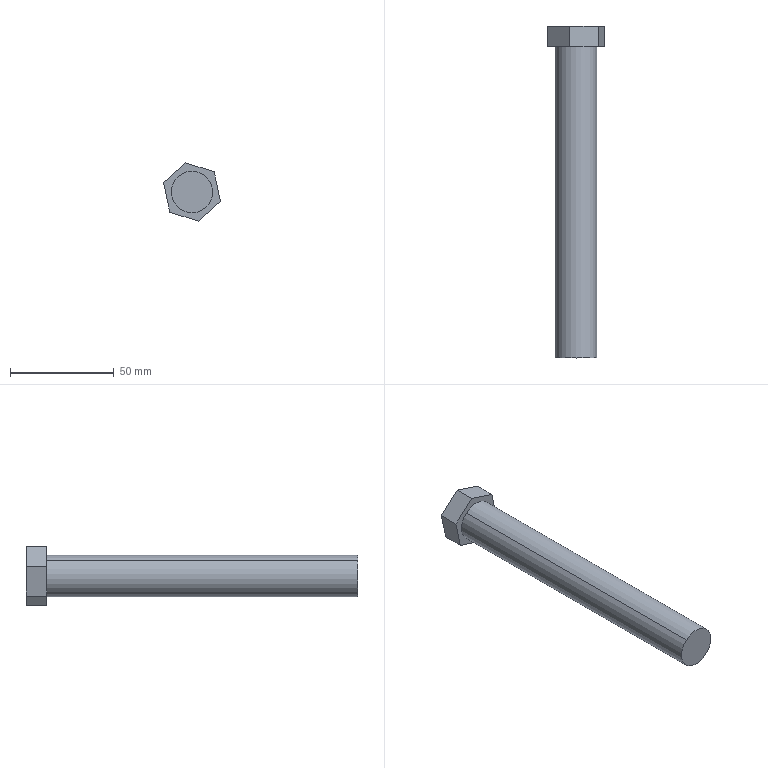Component | SolidWorks | -LimitScrewRod-1 | 1 solid | 11 faces | box 27.46 x 160 x 28.24 mm | volume 52537 mm3 | plane 9 | cylinder 2 | commonest cylinder face diameters 20 x2
STEP:
#1=COLOUR_RGB('',0.7922,0.8196,0.9333);
#2=FILL_AREA_STYLE_COLOUR('',#1);
#3=FILL_AREA_STYLE('',(#2));
#4=SURFACE_STYLE_FILL_AREA(#3);
#5=SURFACE_SIDE_STYLE('',(#4));
#6=SURFACE_STYLE_USAGE(.BOTH.,#5);
#7=PRESENTATION_STYLE_ASSIGNMENT((#6));
#8=CARTESIAN_POINT('',(0.9176,41.772,-4.432));
#9=VERTEX_POINT('',#8);
#10=CARTESIAN_POINT('',(1.445,41.772,-5.017));
#11=VERTEX_POINT('',#10);
#12=CARTESIAN_POINT('',(1.181,41.772,-4.724));
#13=DIRECTION('',(0.,-1.,0.));
#14=DIRECTION('',(-0.6693,0.,0.743));
#15=AXIS2_PLACEMENT_3D('',#12,#13,#14);
#16=CIRCLE('',#15,0.3937);
#17=EDGE_CURVE('',#9,#11,#16,.T.);
#18=ORIENTED_EDGE('',*,*,#17,.F.);
#19=CARTESIAN_POINT('',(0.9176,47.677,-4.432));
#20=VERTEX_POINT('',#19);
#21=CARTESIAN_POINT('',(0.9176,41.772,-4.432));
#22=DIRECTION('',(0.,1.,0.));
#23=VECTOR('',#22,39.37);
#24=LINE('',#21,#23);
#25=EDGE_CURVE('',#9,#20,#24,.T.);
#26=ORIENTED_EDGE('',*,*,#25,.T.);
#27=CARTESIAN_POINT('',(1.445,47.677,-5.017));
#28=VERTEX_POINT('',#27);
#29=CARTESIAN_POINT('',(1.181,47.677,-4.724));
#30=DIRECTION('',(0.,-1.,0.));
#31=DIRECTION('',(-0.6693,0.,0.743));
#32=AXIS2_PLACEMENT_3D('',#29,#30,#31);
#33=CIRCLE('',#32,0.3937);
#34=EDGE_CURVE('',#20,#28,#33,.T.);
#35=ORIENTED_EDGE('',*,*,#34,.T.);
#36=CARTESIAN_POINT('',(1.445,41.772,-5.017));
#37=DIRECTION('',(0.,1.,0.));
#38=VECTOR('',#37,39.37);
#39=LINE('',#36,#38);
#40=EDGE_CURVE('',#11,#28,#39,.T.);
#41=ORIENTED_EDGE('',*,*,#40,.F.);
#42=EDGE_LOOP('',(#18,#26,#35,#41));
#43=FACE_OUTER_BOUND('',#42,.T.);
#44=CARTESIAN_POINT('',(1.181,41.772,-4.724));
#45=DIRECTION('',(0.,1.,0.));
#46=DIRECTION('',(0.6693,0.,-0.743));
#47=AXIS2_PLACEMENT_3D('',#44,#45,#46);
#48=CYLINDRICAL_SURFACE('',#47,0.3937);
#49=ADVANCED_FACE('',(#43),#48,.T.);
#50=CARTESIAN_POINT('',(0.6406,47.677,-4.549));
#51=VERTEX_POINT('',#50);
#52=CARTESIAN_POINT('',(0.7589,47.677,-5.105));
#53=VERTEX_POINT('',#52);
#54=CARTESIAN_POINT('',(0.6406,47.677,-4.549));
#55=DIRECTION('',(0.2081,0.,-0.9781));
#56=VECTOR('',#55,39.37);
#57=LINE('',#54,#56);
#58=EDGE_CURVE('',#51,#53,#57,.T.);
#59=ORIENTED_EDGE('',*,*,#58,.T.);
#60=CARTESIAN_POINT('',(1.299,47.677,-5.28));
#61=VERTEX_POINT('',#60);
#62=CARTESIAN_POINT('',(0.7589,47.677,-5.105));
#63=DIRECTION('',(0.9511,0.,-0.3088));
#64=VECTOR('',#63,39.37);
#65=LINE('',#62,#64);
#66=EDGE_CURVE('',#53,#61,#65,.T.);
#67=ORIENTED_EDGE('',*,*,#66,.T.);
#68=CARTESIAN_POINT('',(1.722,47.677,-4.9));
#69=VERTEX_POINT('',#68);
#70=CARTESIAN_POINT('',(1.299,47.677,-5.28));
#71=DIRECTION('',(0.743,0.,0.6693));
#72=VECTOR('',#71,39.37);
#73=LINE('',#70,#72);
#74=EDGE_CURVE('',#61,#69,#73,.T.);
#75=ORIENTED_EDGE('',*,*,#74,.T.);
#76=CARTESIAN_POINT('',(1.603,47.677,-4.344));
#77=VERTEX_POINT('',#76);
#78=CARTESIAN_POINT('',(1.722,47.677,-4.9));
#79=DIRECTION('',(-0.2081,0.,0.9781));
#80=VECTOR('',#79,39.37);
#81=LINE('',#78,#80);
#82=EDGE_CURVE('',#69,#77,#81,.T.);
#83=ORIENTED_EDGE('',*,*,#82,.T.);
#84=CARTESIAN_POINT('',(1.063,47.677,-4.169));
#85=VERTEX_POINT('',#84);
#86=CARTESIAN_POINT('',(1.603,47.677,-4.344));
#87=DIRECTION('',(-0.9511,0.,0.3088));
#88=VECTOR('',#87,39.37);
#89=LINE('',#86,#88);
#90=EDGE_CURVE('',#77,#85,#89,.T.);
#91=ORIENTED_EDGE('',*,*,#90,.T.);
#92=CARTESIAN_POINT('',(1.063,47.677,-4.169));
#93=DIRECTION('',(-0.743,0.,-0.6693));
#94=VECTOR('',#93,39.37);
#95=LINE('',#92,#94);
#96=EDGE_CURVE('',#85,#51,#95,.T.);
#97=ORIENTED_EDGE('',*,*,#96,.T.);
#98=EDGE_LOOP('',(#59,#67,#75,#83,#91,#97));
#99=FACE_OUTER_BOUND('',#98,.T.);
#100=CARTESIAN_POINT('',(1.181,47.677,-4.724));
#101=DIRECTION('',(0.,-1.,0.));
#102=DIRECTION('',(-0.6693,0.,0.743));
#103=AXIS2_PLACEMENT_3D('',#100,#101,#102);
#104=CIRCLE('',#103,0.3937);
#105=EDGE_CURVE('',#28,#20,#104,.T.);
#106=ORIENTED_EDGE('',*,*,#105,.F.);
#107=ORIENTED_EDGE('',*,*,#34,.F.);
#108=EDGE_LOOP('',(#106,#107));
#109=FACE_BOUND('',#108,.T.);
#110=CARTESIAN_POINT('',(1.181,47.677,-4.724));
#111=DIRECTION('',(0.,-1.,0.));
#112=DIRECTION('',(-0.6693,0.,0.743));
#113=AXIS2_PLACEMENT_3D('',#110,#111,#112);
#114=PLANE('',#113);
#115=ADVANCED_FACE('',(#99,#109),#114,.T.);
#116=CARTESIAN_POINT('',(0.6406,48.071,-4.549));
#117=VERTEX_POINT('',#116);
#118=CARTESIAN_POINT('',(0.7589,48.071,-5.105));
#119=VERTEX_POINT('',#118);
#120=CARTESIAN_POINT('',(0.6406,48.071,-4.549));
#121=DIRECTION('',(0.2081,0.,-0.9781));
#122=VECTOR('',#121,39.37);
#123=LINE('',#120,#122);
#124=EDGE_CURVE('',#117,#119,#123,.T.);
#125=ORIENTED_EDGE('',*,*,#124,.T.);
#126=CARTESIAN_POINT('',(0.7589,47.677,-5.105));
#127=DIRECTION('',(0.,1.,0.));
#128=VECTOR('',#127,39.37);
#129=LINE('',#126,#128);
#130=EDGE_CURVE('',#53,#119,#129,.T.);
#131=ORIENTED_EDGE('',*,*,#130,.F.);
#132=ORIENTED_EDGE('',*,*,#58,.F.);
#133=CARTESIAN_POINT('',(0.6406,47.677,-4.549));
#134=DIRECTION('',(0.,1.,0.));
#135=VECTOR('',#134,39.37);
#136=LINE('',#133,#135);
#137=EDGE_CURVE('',#51,#117,#136,.T.);
#138=ORIENTED_EDGE('',*,*,#137,.T.);
#139=EDGE_LOOP('',(#125,#131,#132,#138));
#140=FACE_OUTER_BOUND('',#139,.T.);
#141=CARTESIAN_POINT('',(0.6406,47.677,-4.549));
#142=DIRECTION('',(0.9781,0.,0.2081));
#143=DIRECTION('',(-0.2081,0.,0.9781));
#144=AXIS2_PLACEMENT_3D('',#141,#142,#143);
#145=PLANE('',#144);
#146=ADVANCED_FACE('',(#140),#145,.F.);
#147=CARTESIAN_POINT('',(1.299,48.071,-5.28));
#148=VERTEX_POINT('',#147);
#149=CARTESIAN_POINT('',(0.7589,48.071,-5.105));
#150=DIRECTION('',(0.9511,0.,-0.3088));
#151=VECTOR('',#150,39.37);
#152=LINE('',#149,#151);
#153=EDGE_CURVE('',#119,#148,#152,.T.);
#154=ORIENTED_EDGE('',*,*,#153,.T.);
#155=CARTESIAN_POINT('',(1.299,47.677,-5.28));
#156=DIRECTION('',(0.,1.,0.));
#157=VECTOR('',#156,39.37);
#158=LINE('',#155,#157);
#159=EDGE_CURVE('',#61,#148,#158,.T.);
#160=ORIENTED_EDGE('',*,*,#159,.F.);
#161=ORIENTED_EDGE('',*,*,#66,.F.);
#162=ORIENTED_EDGE('',*,*,#130,.T.);
#163=EDGE_LOOP('',(#154,#160,#161,#162));
#164=FACE_OUTER_BOUND('',#163,.T.);
#165=CARTESIAN_POINT('',(0.7589,47.677,-5.105));
#166=DIRECTION('',(0.3088,0.,0.9511));
#167=DIRECTION('',(-0.9511,0.,0.3088));
#168=AXIS2_PLACEMENT_3D('',#165,#166,#167);
#169=PLANE('',#168);
#170=ADVANCED_FACE('',(#164),#169,.F.);
#171=CARTESIAN_POINT('',(1.722,48.071,-4.9));
#172=VERTEX_POINT('',#171);
#173=CARTESIAN_POINT('',(1.299,48.071,-5.28));
#174=DIRECTION('',(0.743,0.,0.6693));
#175=VECTOR('',#174,39.37);
#176=LINE('',#173,#175);
#177=EDGE_CURVE('',#148,#172,#176,.T.);
#178=ORIENTED_EDGE('',*,*,#177,.T.);
#179=CARTESIAN_POINT('',(1.722,47.677,-4.9));
#180=DIRECTION('',(0.,1.,0.));
#181=VECTOR('',#180,39.37);
#182=LINE('',#179,#181);
#183=EDGE_CURVE('',#69,#172,#182,.T.);
#184=ORIENTED_EDGE('',*,*,#183,.F.);
#185=ORIENTED_EDGE('',*,*,#74,.F.);
#186=ORIENTED_EDGE('',*,*,#159,.T.);
#187=EDGE_LOOP('',(#178,#184,#185,#186));
#188=FACE_OUTER_BOUND('',#187,.T.);
#189=CARTESIAN_POINT('',(1.299,47.677,-5.28));
#190=DIRECTION('',(-0.6693,0.,0.743));
#191=DIRECTION('',(-0.743,0.,-0.6693));
#192=AXIS2_PLACEMENT_3D('',#189,#190,#191);
#193=PLANE('',#192);
#194=ADVANCED_FACE('',(#188),#193,.F.);
#195=CARTESIAN_POINT('',(1.603,48.071,-4.344));
#196=VERTEX_POINT('',#195);
#197=CARTESIAN_POINT('',(1.722,48.071,-4.9));
#198=DIRECTION('',(-0.2081,0.,0.9781));
#199=VECTOR('',#198,39.37);
#200=LINE('',#197,#199);
#201=EDGE_CURVE('',#172,#196,#200,.T.);
#202=ORIENTED_EDGE('',*,*,#201,.T.);
#203=CARTESIAN_POINT('',(1.603,47.677,-4.344));
#204=DIRECTION('',(0.,1.,0.));
#205=VECTOR('',#204,39.37);
#206=LINE('',#203,#205);
#207=EDGE_CURVE('',#77,#196,#206,.T.);
#208=ORIENTED_EDGE('',*,*,#207,.F.);
#209=ORIENTED_EDGE('',*,*,#82,.F.);
#210=ORIENTED_EDGE('',*,*,#183,.T.);
#211=EDGE_LOOP('',(#202,#208,#209,#210));
#212=FACE_OUTER_BOUND('',#211,.T.);
#213=CARTESIAN_POINT('',(1.722,47.677,-4.9));
#214=DIRECTION('',(-0.9781,0.,-0.2081));
#215=DIRECTION('',(0.2081,0.,-0.9781));
#216=AXIS2_PLACEMENT_3D('',#213,#214,#215);
#217=PLANE('',#216);
#218=ADVANCED_FACE('',(#212),#217,.F.);
#219=CARTESIAN_POINT('',(1.063,48.071,-4.169));
#220=VERTEX_POINT('',#219);
#221=CARTESIAN_POINT('',(1.603,48.071,-4.344));
#222=DIRECTION('',(-0.9511,0.,0.3088));
#223=VECTOR('',#222,39.37);
#224=LINE('',#221,#223);
#225=EDGE_CURVE('',#196,#220,#224,.T.);
#226=ORIENTED_EDGE('',*,*,#225,.T.);
#227=CARTESIAN_POINT('',(1.063,47.677,-4.169));
#228=DIRECTION('',(0.,1.,0.));
#229=VECTOR('',#228,39.37);
#230=LINE('',#227,#229);
#231=EDGE_CURVE('',#85,#220,#230,.T.);
#232=ORIENTED_EDGE('',*,*,#231,.F.);
#233=ORIENTED_EDGE('',*,*,#90,.F.);
#234=ORIENTED_EDGE('',*,*,#207,.T.);
#235=EDGE_LOOP('',(#226,#232,#233,#234));
#236=FACE_OUTER_BOUND('',#235,.T.);
#237=CARTESIAN_POINT('',(1.603,47.677,-4.344));
#238=DIRECTION('',(-0.3088,0.,-0.9511));
#239=DIRECTION('',(0.9511,0.,-0.3088));
#240=AXIS2_PLACEMENT_3D('',#237,#238,#239);
#241=PLANE('',#240);
#242=ADVANCED_FACE('',(#236),#241,.F.);
#243=CARTESIAN_POINT('',(1.063,48.071,-4.169));
#244=DIRECTION('',(-0.743,0.,-0.6693));
#245=VECTOR('',#244,39.37);
#246=LINE('',#243,#245);
#247=EDGE_CURVE('',#220,#117,#246,.T.);
#248=ORIENTED_EDGE('',*,*,#247,.T.);
#249=ORIENTED_EDGE('',*,*,#137,.F.);
#250=ORIENTED_EDGE('',*,*,#96,.F.);
#251=ORIENTED_EDGE('',*,*,#231,.T.);
#252=EDGE_LOOP('',(#248,#249,#250,#251));
#253=FACE_OUTER_BOUND('',#252,.T.);
#254=CARTESIAN_POINT('',(1.063,47.677,-4.169));
#255=DIRECTION('',(0.6693,0.,-0.743));
#256=DIRECTION('',(0.743,0.,0.6693));
#257=AXIS2_PLACEMENT_3D('',#254,#255,#256);
#258=PLANE('',#257);
#259=ADVANCED_FACE('',(#253),#258,.F.);
#260=ORIENTED_EDGE('',*,*,#124,.F.);
#261=ORIENTED_EDGE('',*,*,#247,.F.);
#262=ORIENTED_EDGE('',*,*,#225,.F.);
#263=ORIENTED_EDGE('',*,*,#201,.F.);
#264=ORIENTED_EDGE('',*,*,#177,.F.);
#265=ORIENTED_EDGE('',*,*,#153,.F.);
#266=EDGE_LOOP('',(#260,#261,#262,#263,#264,#265));
#267=FACE_OUTER_BOUND('',#266,.T.);
#268=CARTESIAN_POINT('',(1.181,48.071,-4.724));
#269=DIRECTION('',(0.,-1.,0.));
#270=DIRECTION('',(-0.6693,0.,0.743));
#271=AXIS2_PLACEMENT_3D('',#268,#269,#270);
#272=PLANE('',#271);
#273=ADVANCED_FACE('',(#267),#272,.F.);
#274=ORIENTED_EDGE('',*,*,#25,.F.);
#275=CARTESIAN_POINT('',(1.181,41.772,-4.724));
#276=DIRECTION('',(0.,-1.,0.));
#277=DIRECTION('',(-0.6693,0.,0.743));
#278=AXIS2_PLACEMENT_3D('',#275,#276,#277);
#279=CIRCLE('',#278,0.3937);
#280=EDGE_CURVE('',#11,#9,#279,.T.);
#281=ORIENTED_EDGE('',*,*,#280,.F.);
#282=ORIENTED_EDGE('',*,*,#40,.T.);
#283=ORIENTED_EDGE('',*,*,#105,.T.);
#284=EDGE_LOOP('',(#274,#281,#282,#283));
#285=FACE_OUTER_BOUND('',#284,.T.);
#286=CARTESIAN_POINT('',(1.181,41.772,-4.724));
#287=DIRECTION('',(0.,1.,0.));
#288=DIRECTION('',(0.6693,0.,-0.743));
#289=AXIS2_PLACEMENT_3D('',#286,#287,#288);
#290=CYLINDRICAL_SURFACE('',#289,0.3937);
#291=ADVANCED_FACE('',(#285),#290,.T.);
#292=ORIENTED_EDGE('',*,*,#280,.T.);
#293=ORIENTED_EDGE('',*,*,#17,.T.);
#294=EDGE_LOOP('',(#292,#293));
#295=FACE_OUTER_BOUND('',#294,.T.);
#296=CARTESIAN_POINT('',(1.181,41.772,-4.724));
#297=DIRECTION('',(0.,-1.,0.));
#298=DIRECTION('',(-0.6693,0.,0.743));
#299=AXIS2_PLACEMENT_3D('',#296,#297,#298);
#300=PLANE('',#299);
#301=ADVANCED_FACE('',(#295),#300,.T.);
#302=CLOSED_SHELL('',(#49,#115,#146,#170,#194,#218,#242,#259,#273,#291,#301));
#303=MANIFOLD_SOLID_BREP('',#302);
#304=STYLED_ITEM('',(#7),#303);
#305=PRESENTATION_LAYER_ASSIGNMENT('','',(#304));
#306=(LENGTH_UNIT()NAMED_UNIT(*)SI_UNIT($,.METRE.));
#307=LENGTH_MEASURE_WITH_UNIT(LENGTH_MEASURE(0.0254),#306);
#308=DIMENSIONAL_EXPONENTS(1.,0.,0.,0.,0.,0.,0.);
#309=(CONVERSION_BASED_UNIT('',#307)LENGTH_UNIT()NAMED_UNIT(#308));
#310=UNCERTAINTY_MEASURE_WITH_UNIT(LENGTH_MEASURE(0.00001),#309,'','');
#311=(NAMED_UNIT(*)PLANE_ANGLE_UNIT()SI_UNIT($,.RADIAN.));
#312=(NAMED_UNIT(*)SI_UNIT($,.STERADIAN.)SOLID_ANGLE_UNIT());
#313=(GEOMETRIC_REPRESENTATION_CONTEXT(3)GLOBAL_UNCERTAINTY_ASSIGNED_CONTEXT((#310))GLOBAL_UNIT_ASSIGNED_CONTEXT((#309,#311,#312))REPRESENTATION_CONTEXT('',''));
#314=MECHANICAL_DESIGN_GEOMETRIC_PRESENTATION_REPRESENTATION('',(#304),#313);
#315=CARTESIAN_POINT('',(0.,0.,0.));
#316=DIRECTION('',(0.,0.,1.));
#317=DIRECTION('',(1.,0.,0.));
#318=AXIS2_PLACEMENT_3D('',#315,#316,#317);
#319=(LENGTH_UNIT()NAMED_UNIT(*)SI_UNIT($,.METRE.));
#320=LENGTH_MEASURE_WITH_UNIT(LENGTH_MEASURE(0.0254),#319);
#321=DIMENSIONAL_EXPONENTS(1.,0.,0.,0.,0.,0.,0.);
#322=(CONVERSION_BASED_UNIT('',#320)LENGTH_UNIT()NAMED_UNIT(#321));
#323=UNCERTAINTY_MEASURE_WITH_UNIT(LENGTH_MEASURE(0.00001),#322,'','');
#324=(NAMED_UNIT(*)PLANE_ANGLE_UNIT()SI_UNIT($,.RADIAN.));
#325=(NAMED_UNIT(*)SI_UNIT($,.STERADIAN.)SOLID_ANGLE_UNIT());
#326=(GEOMETRIC_REPRESENTATION_CONTEXT(3)GLOBAL_UNCERTAINTY_ASSIGNED_CONTEXT((#323))GLOBAL_UNIT_ASSIGNED_CONTEXT((#322,#324,#325))REPRESENTATION_CONTEXT('',''));
#327=ADVANCED_BREP_SHAPE_REPRESENTATION('',(#303,#318),#326);